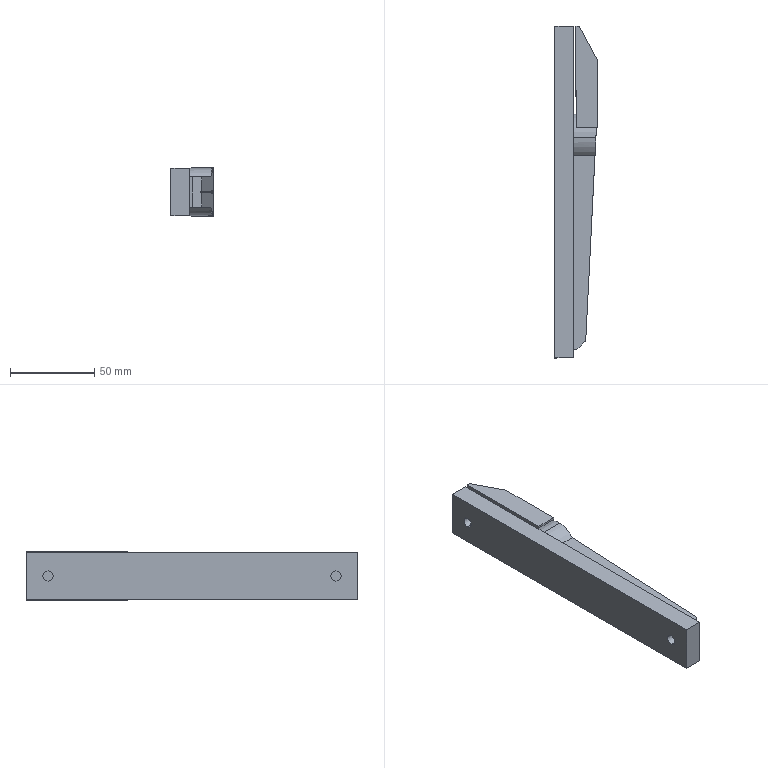Component | SolidWorks | FrontLeftDoor-1_MS830-Lock-1 | 2 solids | 47 faces | volume 104382 mm3 | plane 26 | cylinder 19 | spline 2 | commonest cylinder face diameters 0.5 x11 6 x4 28 x3 29 x1 | material Plain Carbon Steel